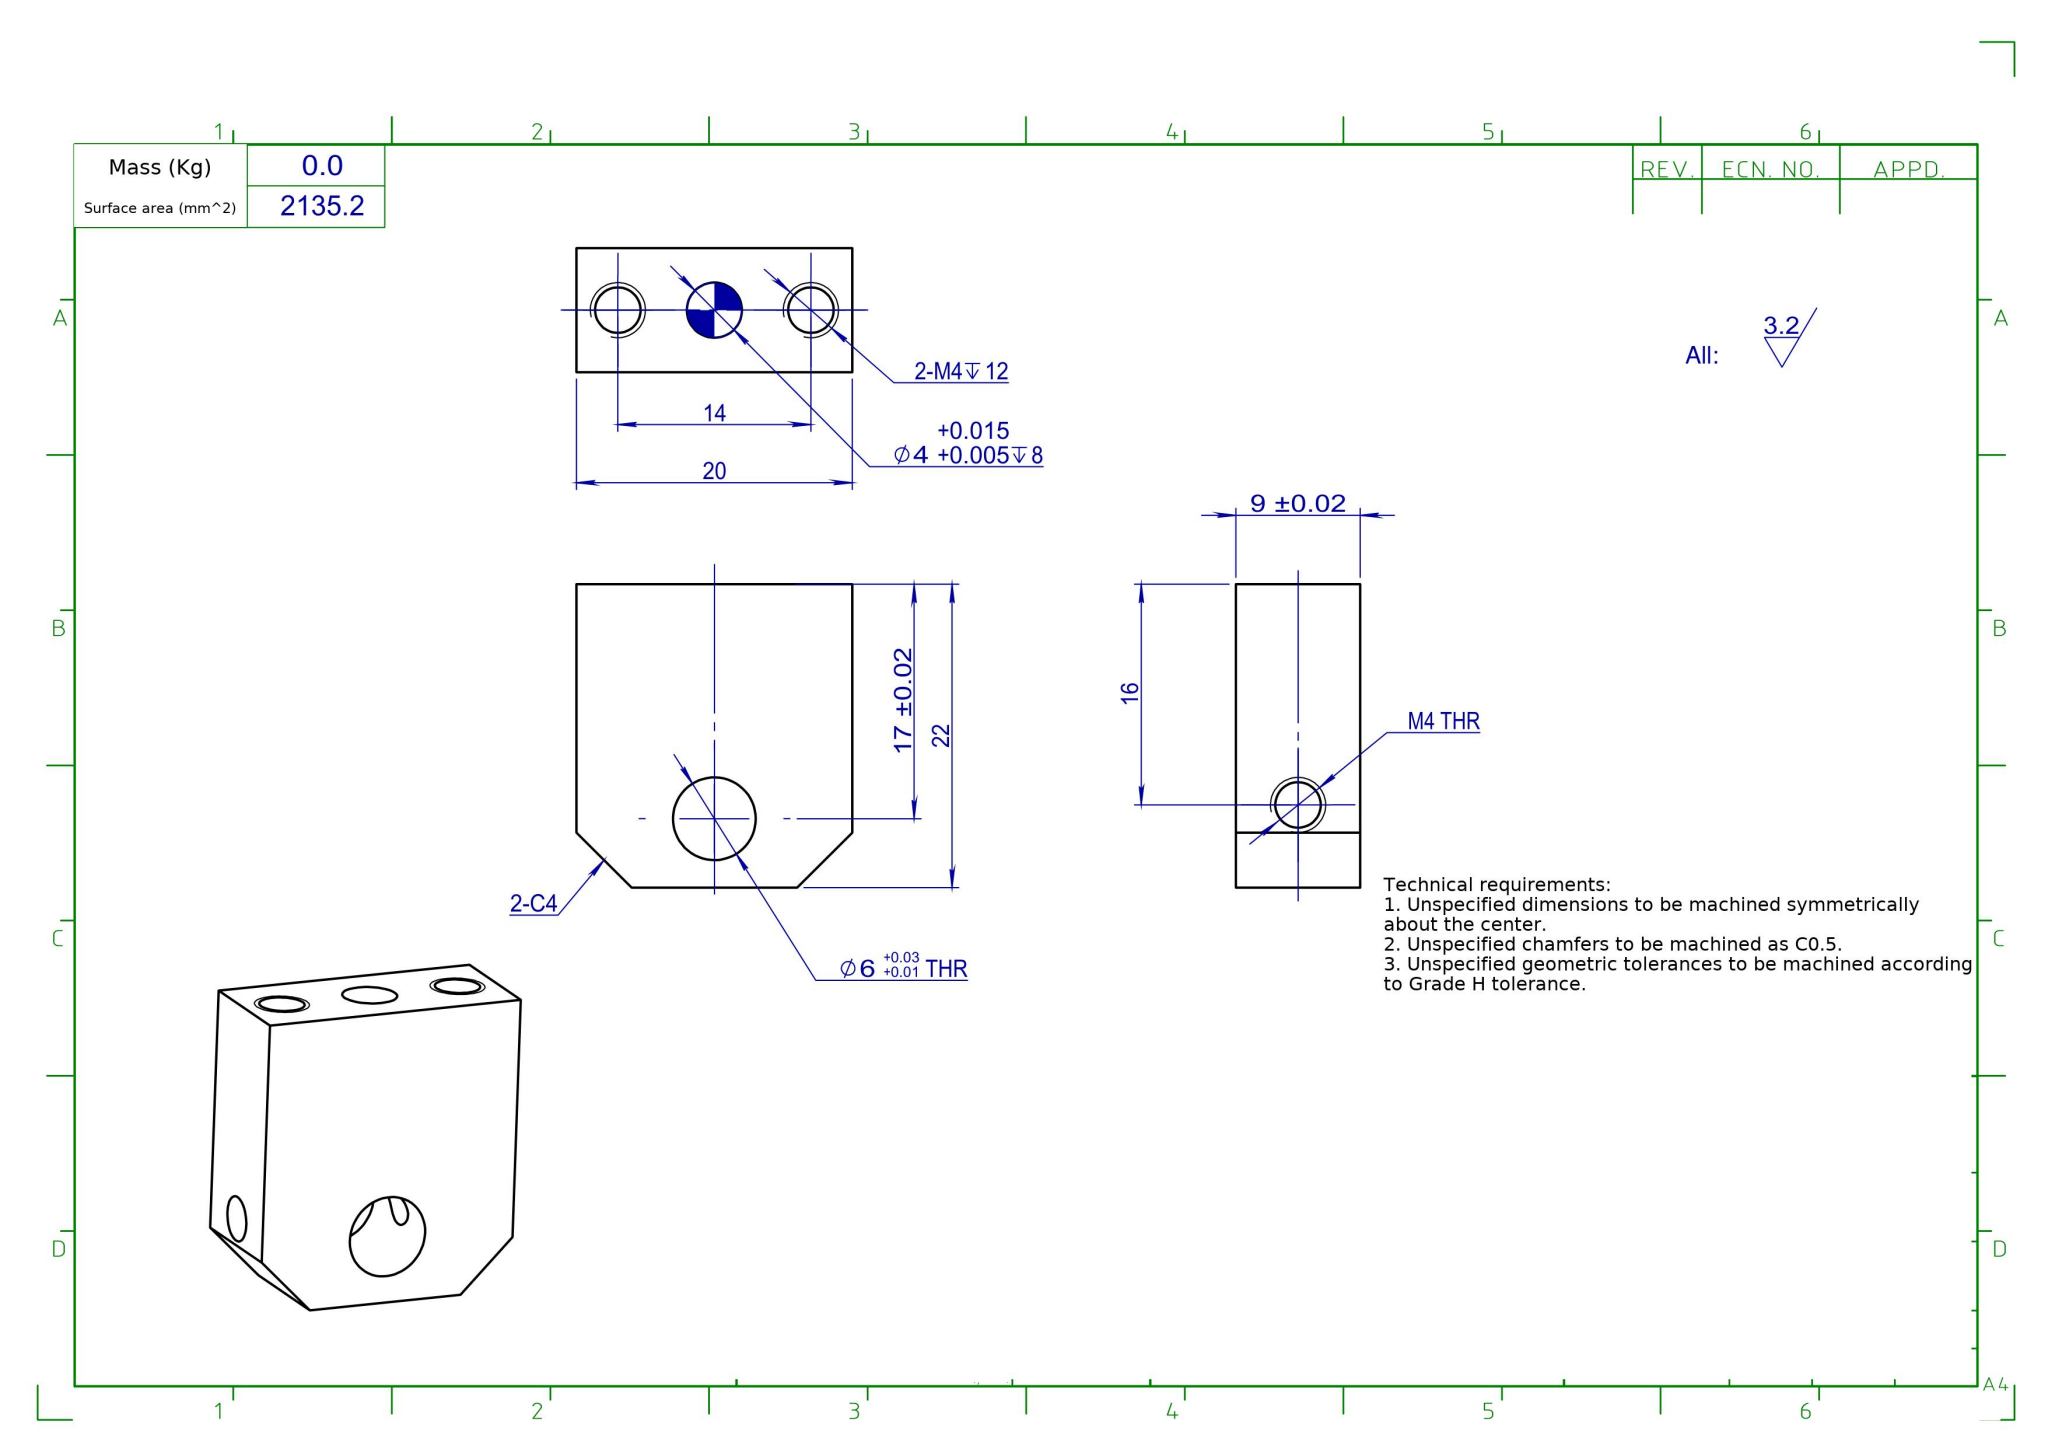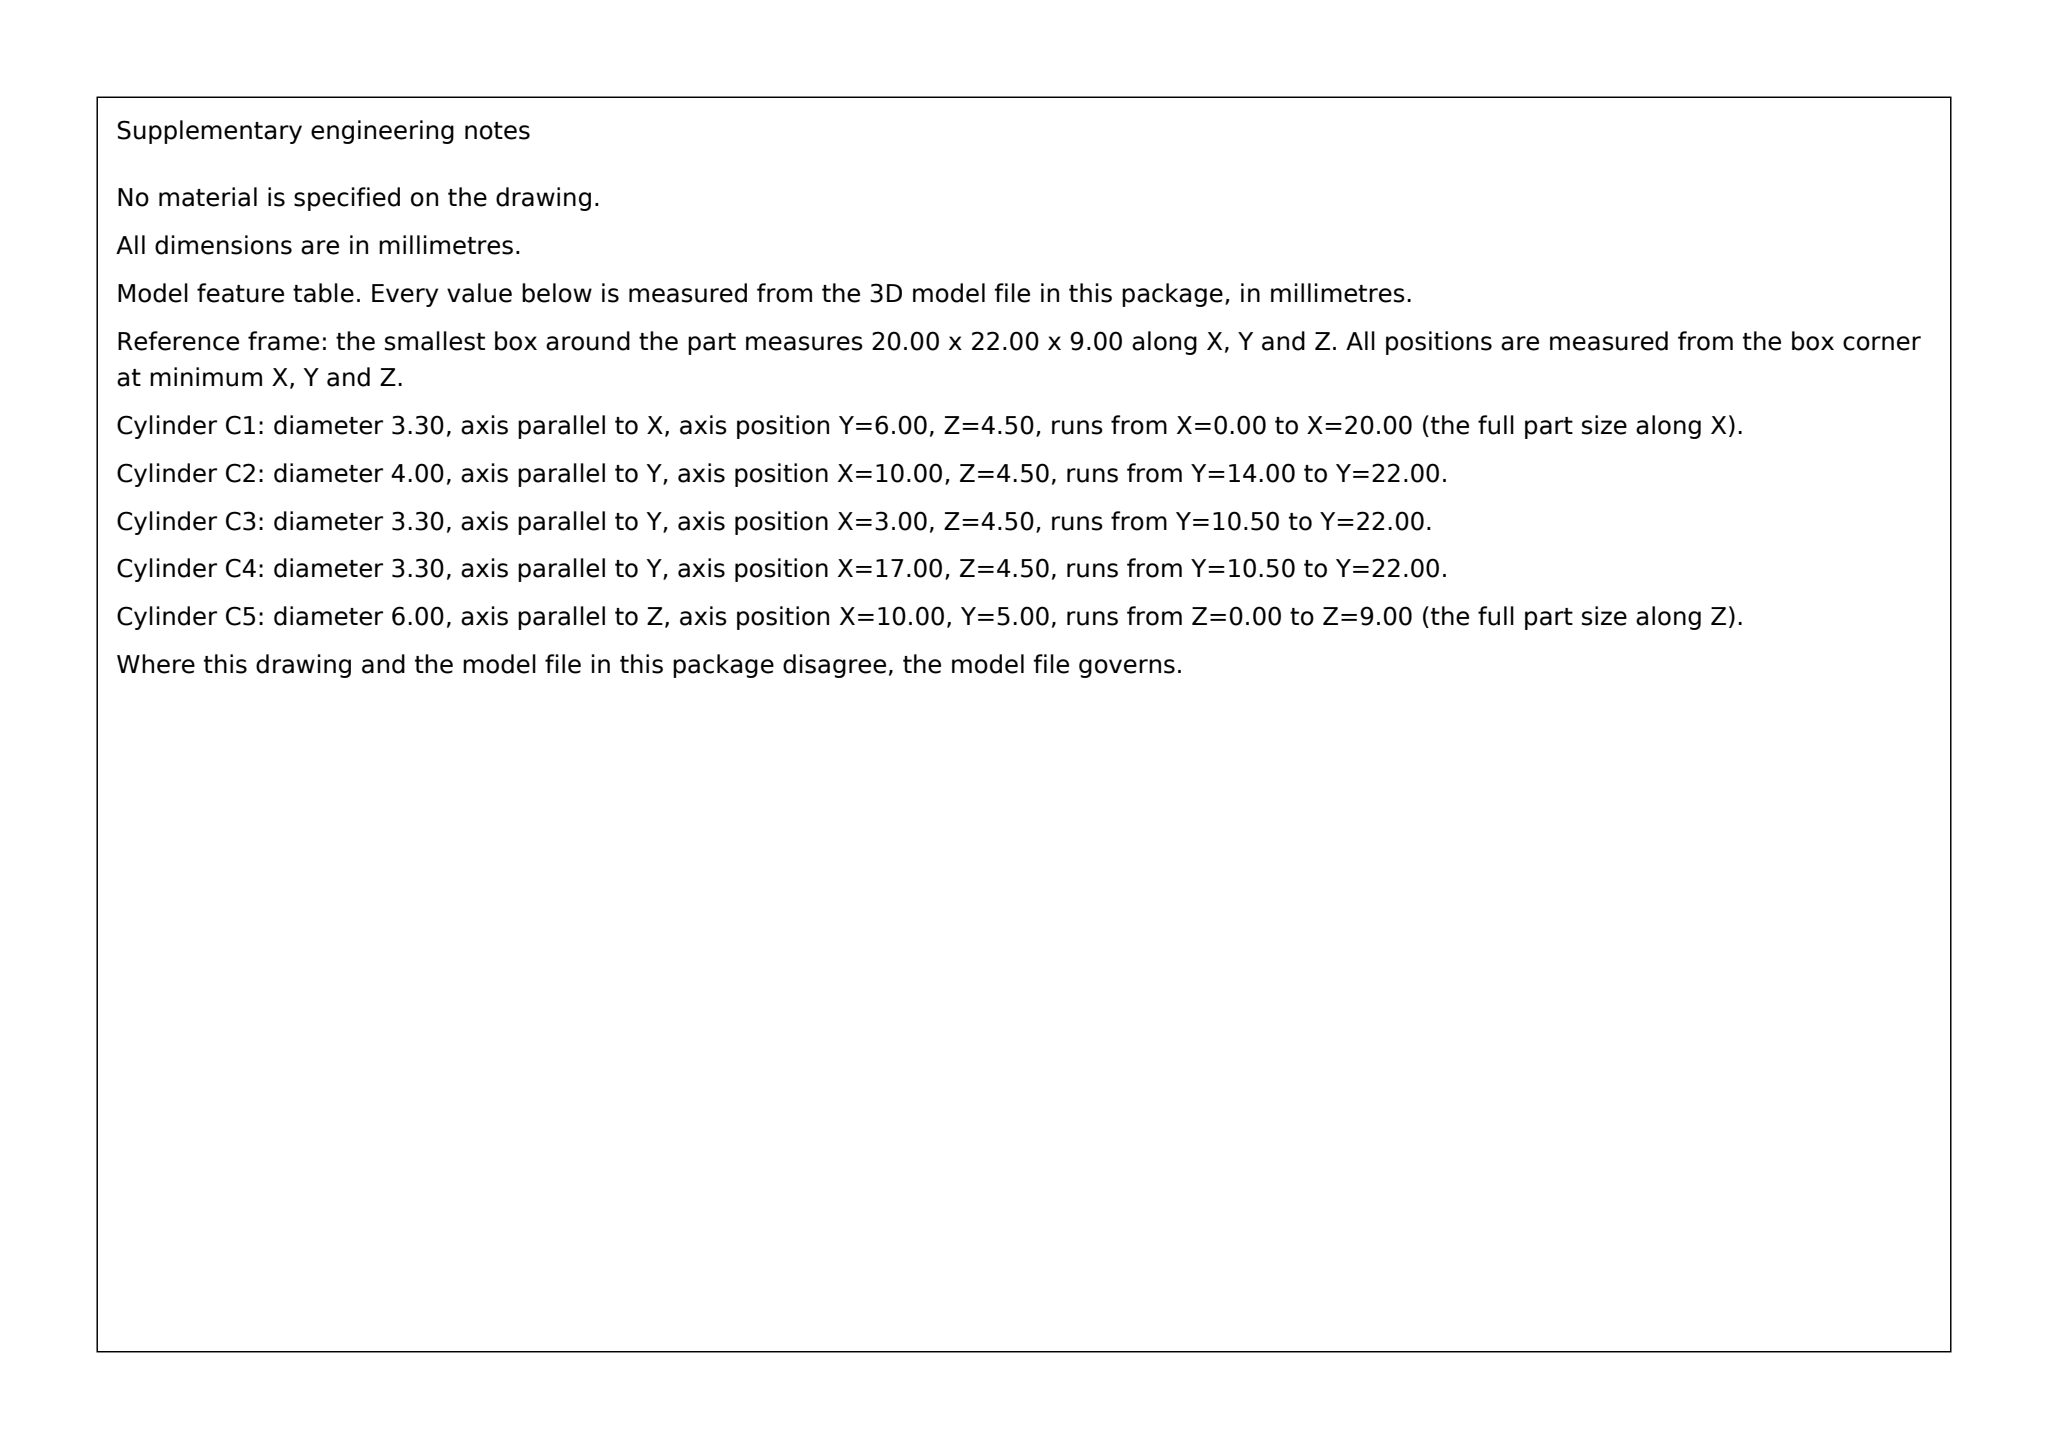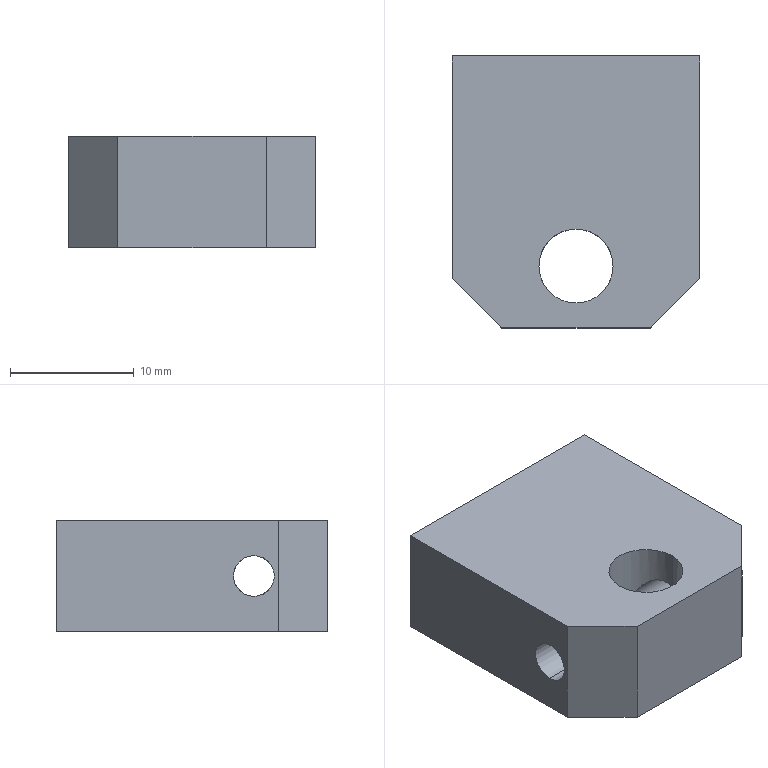Part | SolidWorks | mm | 1 solid | 25 faces | box 20 x 22 x 9 mm | volume 3133 mm3 | cylinder 12 | plane 9 | cone 4 | commonest cylinder face diameters 3.3 x8 4 x2 6 x2
build123d program:
from build123d import *

# Parameters (mm, degrees)
SKETCH1_W             = 20
SKETCH1_H             = 22
EXTRUDE1_DEPTH        = 4.5
SKETCH2_R             = 3
CUT_EXTRUDE1_DEPTH    = 18.378
M4_TAPPED_HOLE1_D     = 3.3
M4_TAPPED_HOLE1_DEPTH = 11.5
M4_TAPPED_HOLE1_TIP   = 0.9914
M4_TAPPED_HOLE2_D     = 3.3
SKETCH10_R            = 2
CUT_EXTRUDE2_DEPTH    = 8
CHAMFER2_SIZE         = 4


with BuildPart() as part:
    # Sketch1 → Extrude1 (new, symmetric)
    with BuildSketch(Plane.XY):
        Rectangle(SKETCH1_W, SKETCH1_H)
    extrude(amount=EXTRUDE1_DEPTH, both=True)

    # Sketch2 → Cut-Extrude1 (cut, through all)
    with BuildSketch(Plane.XY.offset(4.5)):
        with Locations((0, -6)):
            Circle(SKETCH2_R)
    extrude(amount=-CUT_EXTRUDE1_DEPTH, mode=Mode.SUBTRACT)

    # M4 Tapped Hole1
    with Locations(Plane(origin=(0, 11, 0), x_dir=(-1, 0, 0), z_dir=(0, 1, 0))):
        with Locations((7, 0), (-7, 0)):
            Hole(M4_TAPPED_HOLE1_D / 2, depth=M4_TAPPED_HOLE1_DEPTH)
            with Locations((0, 0, -(M4_TAPPED_HOLE1_DEPTH + M4_TAPPED_HOLE1_TIP / 2))):  # 118° drill point
                Cone(0, M4_TAPPED_HOLE1_D / 2, M4_TAPPED_HOLE1_TIP, mode=Mode.SUBTRACT)

    # M4 Tapped Hole2 (through all)
    with Locations(Plane(origin=(10, 0, 0), x_dir=(0, 0, -1), z_dir=(1, 0, 0))):
        with Locations((0, -5)):
            Hole(M4_TAPPED_HOLE2_D / 2)

    # Sketch10 → Cut-Extrude2 (cut)
    with BuildSketch(Plane(origin=(0, 11, 0), x_dir=(1, 0, 0), z_dir=(0, 1, 0))):
        with Locations(Location((0, 0, 0), (0, 0, 270))):
            Circle(SKETCH10_R)
    extrude(amount=-CUT_EXTRUDE2_DEPTH, mode=Mode.SUBTRACT)

    # Chamfer2
    chamfer2_edges = [part.edges().sort_by_distance(p)[0] for p in [
        (10, -11, 0),
        (-10, -11, 0),
    ]]
    chamfer(chamfer2_edges, length=CHAMFER2_SIZE)


solid = part.part